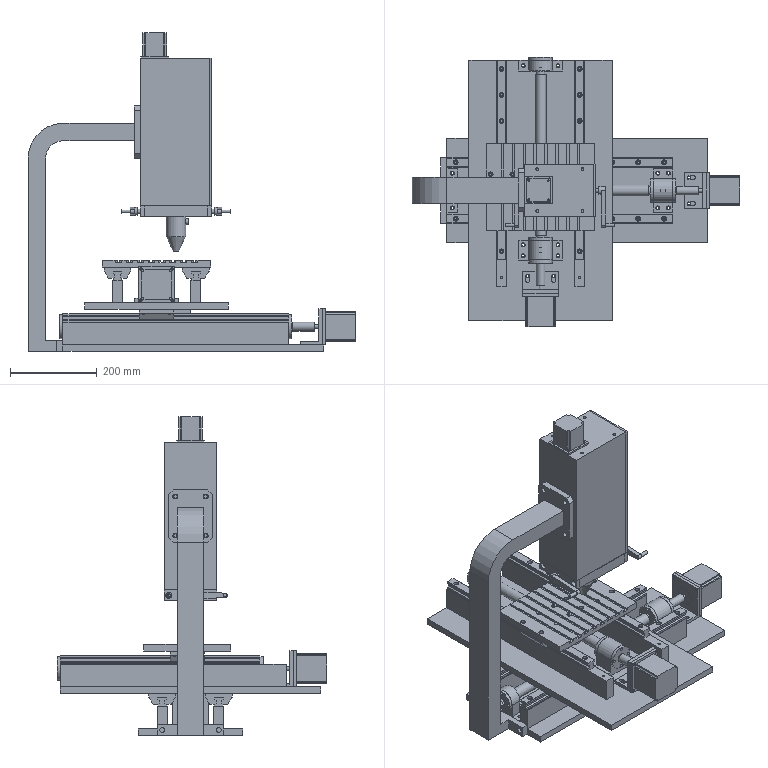Assembly | NX | mm | 67 component files | 122 solids | 1525 faces | box 754 x 621 x 734 mm | volume 16256639 mm3 | plane 882 | cylinder 528 | cone 51 | sphere 48 | torus 16 | commonest cylinder face diameters 5 x100 7 x62 11 x60 6.8 x36 9 x36 6 x28 35 x24 8 x14
Bill of materials:
unnamed part 1 | 1 |  | Bar with a rectangular cross-section bent into a C/J shape, with one rounded 90-degree bend. One end has a square plate flange with chamfered corners and four corner holes. The other end has a narrow rectangular tab flange with two holes.
unnamed part 2 | 1 |  | Thick plate-and-boss block. A straight rectangular plate is joined to a round-ended body that has a large vertical through-bore, with a stepped inner lip in the bore. Four small holes sit around the bore on the top face.
unnamed part 3 | 1 |  | Solid block with one semicircular rounded end, shaped like a D in plan. A vertical through-hole passes near the rounded end. The flat end face opposite the round has four small holes in a rectangular pattern.
unnamed part 4 | 2 |  | Crank-like arm. A tapered flat link has a round boss with a through-hole at its wide end and a cylindrical pin sticking out perpendicular at its narrow, rounded end.
unnamed part 5 | 2 |  | Circular flange disc with a raised concentric circular boss. The boss has a shallow recess with a sloped or chamfered wall and a central through-hole. Four through-holes are spaced evenly around the outer flange ring.
unnamed part 6 | 1 |  | Tall rectangular box-like frame or enclosure with one long side open. The top and bottom plates have one larger hole and several small holes. Small holes are visible at the corners of the open edges.
unnamed part 7 | 2 |  | Short solid cylinder, like a thick washer or spacer, with a central through-hole and rounded or filleted outer edges.
unnamed part 8 | 2 |  | Upright with a rounded top and a large horizontal through-bore, on a rectangular base plate that extends on both sides. Each extension has one vertical through-hole. Overall it resembles a pillow-block-style support.
unnamed part 9 | 1 |  | Vertical cylinder with a shallow recess at the top rim and a cone-shaped lower end with a small flat at the bottom. A short cylindrical pin sticks out radially from the side wall.
unnamed part 10 | 2 |  | Long cylindrical tube or sleeve with a circular flange at one end. The flange has four evenly spaced bolt-type holes and a large central bore.
unnamed part 11 | 1 |  | Square prismatic body with concave grooves running along all four vertical edges. It sits on a thin square plate that overhangs it and has four corner through-holes. Below the plate there is a short cylindrical boss and a smaller cylindrical shaft sticking out.
unnamed part 12 | 1 |  | Long slender rectangular bar. One end has a thicker rectangular head with four holes. The other end has a thin disc-like foot with a flat cut on one side.
unnamed part 13 | 1 |  | Prismatic extrusion with a thin flat flange plate along one side and a round-ended boss with a large through-bore; profile looks like a 'P' or 'b' in plan.
unnamed part 14 | 4 |  | Circular flange disc with a large central bore, four equally spaced through holes on a bolt circle, and a short low cylindrical spigot/register on one face.
unnamed part 15 | 1 |  | Long, slender, solid turned shaft with several stepped diameters: a largest central section, then progressively smaller steps toward both ends.
unnamed part 16 | 1 |  | Rectangular flat plate with eight parallel T-slots running across the top face and a pattern of through holes.
unnamed part 17 | 2 |  | Square-section boxy body with a square mounting flange on one end that has four corner holes; a cylindrical pilot boss and a smaller protruding round shaft stick out from the flange face.
unnamed part 18 | 2 |  | Block with a flat rectangular top and a semicircular rounded bottom, a large through bore along its length, four holes on the top face, and four holes on the end face around the bore.
unnamed part 19 | 2 |  | Flanged bushing: circular flange with four equally spaced through holes and a longer cylindrical hub with a central through bore.
unnamed part 20 | 2 |  | Long straight rail with a constant waisted (dog-bone-like) cross-section, chamfered top corners, and a row of evenly spaced counterbored vertical holes along its length.
unnamed part 21 | 2 |  | Long straight rail with a waisted cross-section and chamfered corners, and a row of evenly spaced counterbored vertical holes; same profile family as the other rail.
unnamed part 22 | 1 |  | Plain cylindrical tube/spacer with a concentric through bore and flat ends.
unnamed part 23 | 2 |  | Thin flat annular washer-like ring with a central through hole.
unnamed part 24 | 1 |  | Two separate, mirrored rectangular bar bodies, each with a lengthwise notch/groove on its inner side, two vertical through holes, and a small hole in the end face.
unnamed part 25 | 1 |  | Long, slender, solid stepped cylindrical shaft. It has a long uniform main section, short steps at one end, and a run of several smaller steps at the other end that narrows to a small tip.
unnamed part 26 | 2 |  | Rectangular bar with three round through-holes in a row along its length, passing through the wide face.
unnamed part 27 | 1 |  | Flat rectangular base plate with two parallel raised rectangular ribs running along most of its length. Rows of small holes run along the top of each rib, and a group of small holes sits in the plate near one end.
unnamed part 28 | 1 |  | Flat rectangular base plate with two parallel raised rectangular ribs running along most of its length. Small holes run along the rib tops, and a cluster of small holes sits in the plate near one end.
unnamed part 29 | 2 |  | Prismatic block with a V-shaped notch cut into one long side and a T-shaped slot cut into the opposite side. The cuts run through the full height.
unnamed part 30 | 2 |  | Thin-walled cylindrical ring or short tube with plain cylindrical inner and outer surfaces.
unnamed part 31 | 2 |  | L-shaped angle bracket. The upright plate has a large central round hole and four small holes near its corners. The base flange has two parallel elongated slots.
unnamed part 32 | 2 |  | Thick-walled cylindrical tube or spacer with a concentric through-bore and plain outer surface.
unnamed part 33 | 2 |  | Solid stepped cylindrical pin or shaft. A larger-diameter section is at one end, a long middle section follows, and a narrow groove separates a short end section at the opposite end.
unnamed part 34 | 1 |  | Long, slender, solid stepped cylindrical shaft. It has a uniform main body, a few short steps at one end, and several steps at the other end that narrow to a small tip.
GB-T292_AC-1994,7202_AC | 6 |  | Annular ring assembly shaped like an open (unshielded) radial ball bearing: two concentric rings, outer and inner, with a single row of eight spheres spaced evenly in the annular gap between them, and a through-bore in the middle.
unnamed part 35 | 2 |  | Pillow-block-style housing. A rectangular base plate with four through-holes, two on each side, supports an upright body with a rounded top. The body has a large horizontal through-bore and four small holes around the bore on one face.
unnamed part 36 | 4 |  | Rectangular carriage-like block. It has a flat top with four holes near the corners, angled lower sides, and a stepped, T-like channel running along its length on the underside.
unnamed part 37 | 1 |  | Thin flat rectangular plate, tall and narrow (roughly 1:2.8 width-to-height in the face view), with four small round holes, one near each corner.
Mates:
1. fix | glue_arm 1 component
2. concentric | Z_axis_housing 1 edge | glue_arm 1 edge
3. touch align | glue_arm 1 face | Z_axis_housing 1 face
4. touch align | Z_axis_leadscrew 1 face | Z_axis_housing 1 face
5. concentric | Z_axis_leadscrew_nut 1 edge | press_body 1 edge
6. touch align | Z_axis_leadscrew_nut 1 face | Z_axis_leadscrew 1 face
7. concentric | bearing_8_34 2 edge | bearing_block 1 edge
8. concentric | bearing_cover 2 edge | bearing_block 1 edge
9. touch align | bearing_cover 2 face | bearing_block 1 face
10. touch align | bearing_cover 2 face | Z_axis_leadscrew 1 face
11. distance | Z_axis_leadscrew_nut 1 face | bearing_block 1 face
12. distance | Z_axis_leadscrew 1 face | bearing_cover 2 face
13. distance | Z_axis_leadscrew_nut 1 face | Z_axis_housing 1 face
14. concentric | bearing_8_34 1 edge | bearing_block_2 1 edge
15. touch align | bearing_cover 1 face | bearing_block_2 1 face
16. concentric | bearing_cover 1 edge | bearing_block_2 1 edge
17. distance | bearing_block_2 1 face | Z_axis_leadscrew_nut 1 face
18. concentric | glue_stick 1 edge | Z_axis_housing 1 edge
19. concentric | fixture_mount 2 edge | fixture 1 edge
20. touch align | fixture_mount 2 face | fixture 1 face
21. concentric | fixture_mount 1 edge | fixture 1 edge
22. touch align | V_block 2 face | glue_stick 1 face
23. touch align | V_block 2 face | glue_stick 1 face
24. center | V_block 2 face | V_block 2 face | fixture 1 face | fixture 1 face
25. touch align | threaded_rod 2 face | fixture_mount 1 face
26. touch align | threaded_rod 2 face | V_block 2 face
27. center | V_block 2 face | V_block 2 face | fixture_mount 1 face | fixture_mount 1 face
28. touch align | fixture_mount 1 face | Z_axis_housing 1 face
29. touch align | fixture 1 face | Z_axis_housing 1 face
30. touch align | V_block 1 face | glue_stick 1 face
31. touch align | V_block 1 face | glue_stick 1 face
32. touch align | threaded_rod 1 face | fixture_mount 2 face
33. touch align | threaded_rod 1 face | V_block 1 face
34. concentric | housing_cover 1 edge | Z_axis_housing 1 edge
35. touch align | housing_cover 1 face | Z_axis_housing 1 face
36. touch align | guide_rail_base_2 1 face | glue_arm 1 face
37. touch align | guide_rail_base_2 1 face | glue_arm 1 face
38. center | guide_rail_base_2 1 face | guide_rail_base_2 1 face | glue_arm 1 face | glue_arm 1 face
39. concentric | bearing_block_3 2 edge | guide_rail_base_2 1 edge
40. touch align | bearing_block_3 2 face | guide_rail_base_2 1 face
41. concentric | GB-T292_AC-1994_7202_AC 6 edge | bearing_block_3 2 edge
42. touch align | bearing_end_cap 2 face | bearing_block_3 2 face
43. concentric | bearing_end_cap 2 edge | bearing_block_3 2 edge
44. concentric | X_leadscrew 1 edge | GB-T292_AC-1994_7202_AC 6 edge
45. concentric | retaining_ring 2 edge | GB-T292_AC-1994_7202_AC 5 edge
46. concentric | GB-T292_AC-1994_7202_AC 4 edge | retaining_ring 2 edge
47. concentric | bushing 2 edge | GB-T292_AC-1994_7202_AC 4 edge
48. touch align | bearing_block_4 2 face | bushing 2 face
49. touch align | bearing_end_cap_2 4 face | bearing_block_4 2 face
50. concentric | bearing_end_cap_2 4 edge | bearing_block_4 2 edge
51. concentric | GB-T292_AC-1994_7202_AC 5 edge | bearing_end_cap_2 4 edge
52. touch align | bearing_end_cap_2 3 face | bearing_block_4 2 face
53. concentric | bearing_end_cap_2 3 edge | bearing_block_4 2 edge
54. concentric | bearing_block_4 2 edge | guide_rail_base_2 1 edge
55. concentric | motor_bracket 2 edge | guide_rail_base_2 1 edge
56. touch align | linear_guide_rail_2 2 face | guide_rail_base_2 1 face
57. concentric | linear_guide_rail_2 2 edge | guide_rail_base_2 1 edge
58. bond | guide_rail_base_2 1 component | assembly component
59. bond | linear_guide_rail_2 2 component | assembly component
60. bond | linear_guide_rail_2 1 component | assembly component
61. linear | assembly datumaxis | assembly cartesiancoordinatesystem | assembly cartesiancoordinatesystem
62. concentric | handle 2 edge | threaded_rod 2 edge
63. concentric | handle 1 edge | threaded_rod 1 edge
64. center | linear_slider 4 face | linear_slider 4 face | linear_guide_rail_2 2 face | linear_guide_rail_2 2 face
65. touch align | linear_slider 4 face | linear_guide_rail_2 2 face
66. distance | linear_slider 4 face | linear_guide_rail_2 2 face
67. bond | linear_slider 4 component | assembly component
68. bond | linear_slider 3 component | assembly component
69. linear | assembly datumaxis | assembly cartesiancoordinatesystem | assembly cartesiancoordinatesystem
70. touch align | guide_rail_base 1 face | linear_slider 4 face
71. center | guide_rail_base 1 face | guide_rail_base 1 face | linear_slider 4 face | linear_slider 4 face
72. distance | guide_rail_base 1 face | guide_rail_base_2 1 face
73. concentric | motor_bracket 1 edge | guide_rail_base 1 edge
74. concentric | bearing_block_3 1 edge | guide_rail_base 1 edge
75. concentric | GB-T292_AC-1994_7202_AC 2 edge | bearing_block_3 1 edge
76. concentric | bearing_end_cap 1 edge | bearing_block_3 1 edge
77. concentric | Y_leadscrew 1 edge | GB-T292_AC-1994_7202_AC 2 edge
78. concentric | bearing_block_4 1 edge | guide_rail_base 1 edge
79. concentric | bearing_end_cap_2 1 edge | GB-T292_AC-1994_7202_AC 3 edge
80. concentric | retaining_ring 1 edge | GB-T292_AC-1994_7202_AC 3 edge
81. concentric | GB-T292_AC-1994_7202_AC 1 edge | retaining_ring 1 edge
82. concentric | bushing 1 edge | GB-T292_AC-1994_7202_AC 1 edge
83. concentric | bearing_end_cap_2 2 edge | bushing 1 edge
84. concentric | bearing_end_cap_2 1 edge | bearing_block_4 1 edge
85. concentric | linear_cutter_rail 2 edge | guide_rail_base 1 edge
86. parallel | linear_cutter_rail 2 face | guide_rail_base 1 face
87. bond | guide_rail_base 1 component | assembly component
88. bond | linear_cutter_rail 2 component | assembly component
89. bond | linear_cutter_rail 1 component | assembly component
90. linear | assembly datumaxis | assembly cartesiancoordinatesystem | assembly cartesiancoordinatesystem
91. center | linear_slider 2 face | linear_slider 2 face | linear_cutter_rail 2 face | linear_cutter_rail 2 face
92. touch align | linear_slider 2 face | linear_cutter_rail 2 face
93. distance | linear_slider 2 face | linear_cutter_rail 2 face
94. bond | linear_slider 2 component | assembly component
95. bond | linear_slider 1 component | assembly component
96. linear | assembly datumaxis | assembly cartesiancoordinatesystem | assembly cartesiancoordinatesystem
97. touch align | leadscrew_nut 1 face | sleeve 1 face
98. concentric | leadscrew_nut 1 edge | sleeve 1 edge
99. touch align | leadscrew_nut 1 face | X_leadscrew 1 face
100. distance | leadscrew_nut 1 face | guide_rail_base 1 face
101. touch align | leadscrew_nut 2 face | sleeve 2 face
102. concentric | leadscrew_nut 2 edge | sleeve 2 edge
103. concentric | sleeve 2 edge | workbench 1 edge
104. concentric | workbench 1 edge | linear_slider 2 edge
105. concentric | motor_1 1 edge | Z_axis_housing 1 edge
106. concentric | motor_2 2 edge | motor_bracket 2 edge
107. touch align | coupling_2 2 face | X_leadscrew 1 face
108. distance | coupling_2 2 face | bearing_end_cap_2 3 face
109. touch align | coupling 1 face | motor_1 1 face
110. distance | coupling 1 face | bearing_cover 2 face
111. concentric | motor_2 1 edge | motor_bracket 1 edge
112. distance | coupling_2 1 face | bearing_end_cap_2 2 face
113. touch align | coupling_2 1 face | Y_leadscrew 1 face